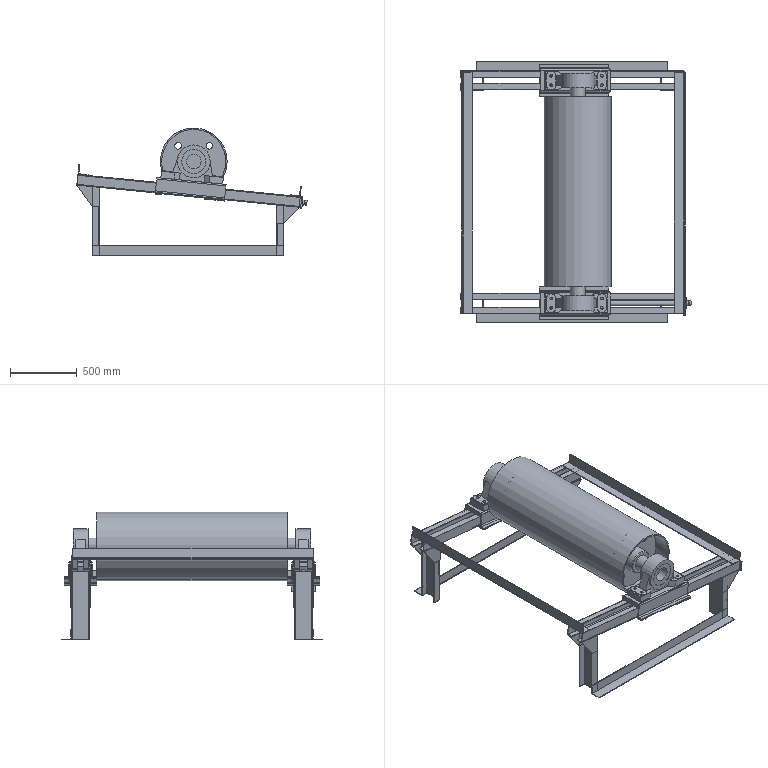Assembly | NX | mm | 35 component files | 36 solids | 384 faces | box 1720.64 x 1950 x 955.84 mm | volume 81203000 mm3 | plane 312 | cylinder 64 | other 4 | cone 4 | commonest cylinder face diameters 20 x16 70 x8 50 x8 180 x6 110 x5 10 x4 34 x4 6 x4
Bill of materials:
unnamed part 1 | 4 |  | Thin flat plate with a four-sided irregular outline: two adjacent straight edges at roughly a right angle, one long slanted edge and a nearly straight top edge; uniform thickness.
unnamed part 2 | 1 |  | Long, slender, solid round rod. One end has a short reduced or faceted section; the end view shows flats or a pointed faceted profile.
unnamed part 3 | 4 |  | Thin flat plate with a four-sided outline: one straight vertical edge, a short bottom edge, a long slanted edge and a near-horizontal top edge; uniform thickness.
unnamed part 4 | 2 |  | Straight thin-walled C/U-channel with a flat web, two parallel flanges and sharp corners.
unnamed part 5 | 1 |  | Rectangular flat plate with one circular through-hole near the center.
unnamed part 6 | 1 |  | Solid circular rod or pin with plain flat ends and constant diameter.
unnamed part 7 | 2 |  | Long rectangular flat bar or strip of uniform thin thickness.
unnamed part 8 | 2 |  | Long straight angle (L-section) profile with thin legs of roughly similar length and a sharp inside corner.
unnamed part 9 | 2 |  | Long straight angle (L-section) profile with roughly equal legs and a relatively thicker wall than a thin sheet angle.
unnamed part 10 | 2 |  | Straight hat-section (omega) profile: raised flat top, two vertical walls and two outward flat flanges, with rounded bends.
unnamed part 11 | 1 |  | Hollow cylindrical tube with an internal end disc recessed inside one end. The disc has a central raised boss with a bore and four smaller holes in a square pattern.
unnamed part 12 | 2 |  | Rectangular flat plate of uniform thickness with no visible holes or cutouts.
unnamed part 13 | 2 |  | Plain thin rectangular flat plate or bar with no visible holes or cutouts.
unnamed part 14 | 4 |  | Long, slender straight member with a thin-walled C/channel-type open cross-section.
unnamed part 15 | 1 |  | Square flat plate with one large central through-hole and four smaller through-holes, one near each corner, in a symmetric pattern.
unnamed part 16 | 2 |  | Short, straight, thin-walled channel (C-section) with a wide web, two parallel flanges, and an open side.
unnamed part 17 | 2 |  | Housing that looks like a pillow block: a cylindrical boss with a central through-bore sits on a tapered pedestal, with a rectangular foot on each side; each foot has two small through-holes.
Mates:
1. fix | down_frame1430 2 component
2. fix | down_frame1430 2 component
3. fix | left_frame600 2 component
4. fix | down_frame1430 2 component
5. fix | right_frame450 2 component
6. touch align | up_frame1670 3 face | right_frame450 2 face
7. touch align | up_frame1670 3 face | up_frame1670 4 face
8. touch align | up_right_frame1800 2 face | up_frame1670 4 face
9. touch align | up_right_frame1800 2 face | up_frame1670 4 face
10. touch align | up_right_frame1800 2 face | up_frame1670 4 face
11. touch align | up_right_frame1800 1 face | up_frame1670 4 face
12. touch align | up_right_frame1800 1 face | up_frame1670 4 face
13. touch align | up_right_frame1800 1 face | up_frame1670 4 face
14. distance | moving_frame 2 face | up_frame1670 4 face
15. touch align | moving_frame_block_1 2 face | up_frame1670 3 face
16. touch align | moving_frame_block_1 2 face | moving_frame 2 face
17. distance | right_frame450 2 face | up_frame1670 4 face
18. distance | up_frame1670 3 face | right_frame450 2 face
19. distance | moving_frame 2 face | up_frame1670 3 face
20. touch align | moving_frame_block_1 2 face | up_frame1670 4 face
21. touch align | moving_frame_block_2 2 face | moving_frame 2 face
22. touch align | moving_frame_block_2 2 face | moving_frame 2 face
23. touch align | moving_frame_block_2 2 face | moving_frame 2 face
24. touch align | moving_frame_block_3 2 face | moving_frame 2 face
25. touch align | moving_frame_block_3 2 face | moving_frame 2 face
26. touch align | moving_frame_block_3 2 face | moving_frame 2 face
27. touch align | up_frame_block_1 1 face | up_frame1670 4 face
28. touch align | up_frame_block_1 1 face | up_frame1670 4 face
29. touch align | up_frame_block_1 1 face | up_frame_block_2 1 face
30. touch align | up_frame_block_1 1 face | up_frame_block_2 1 face